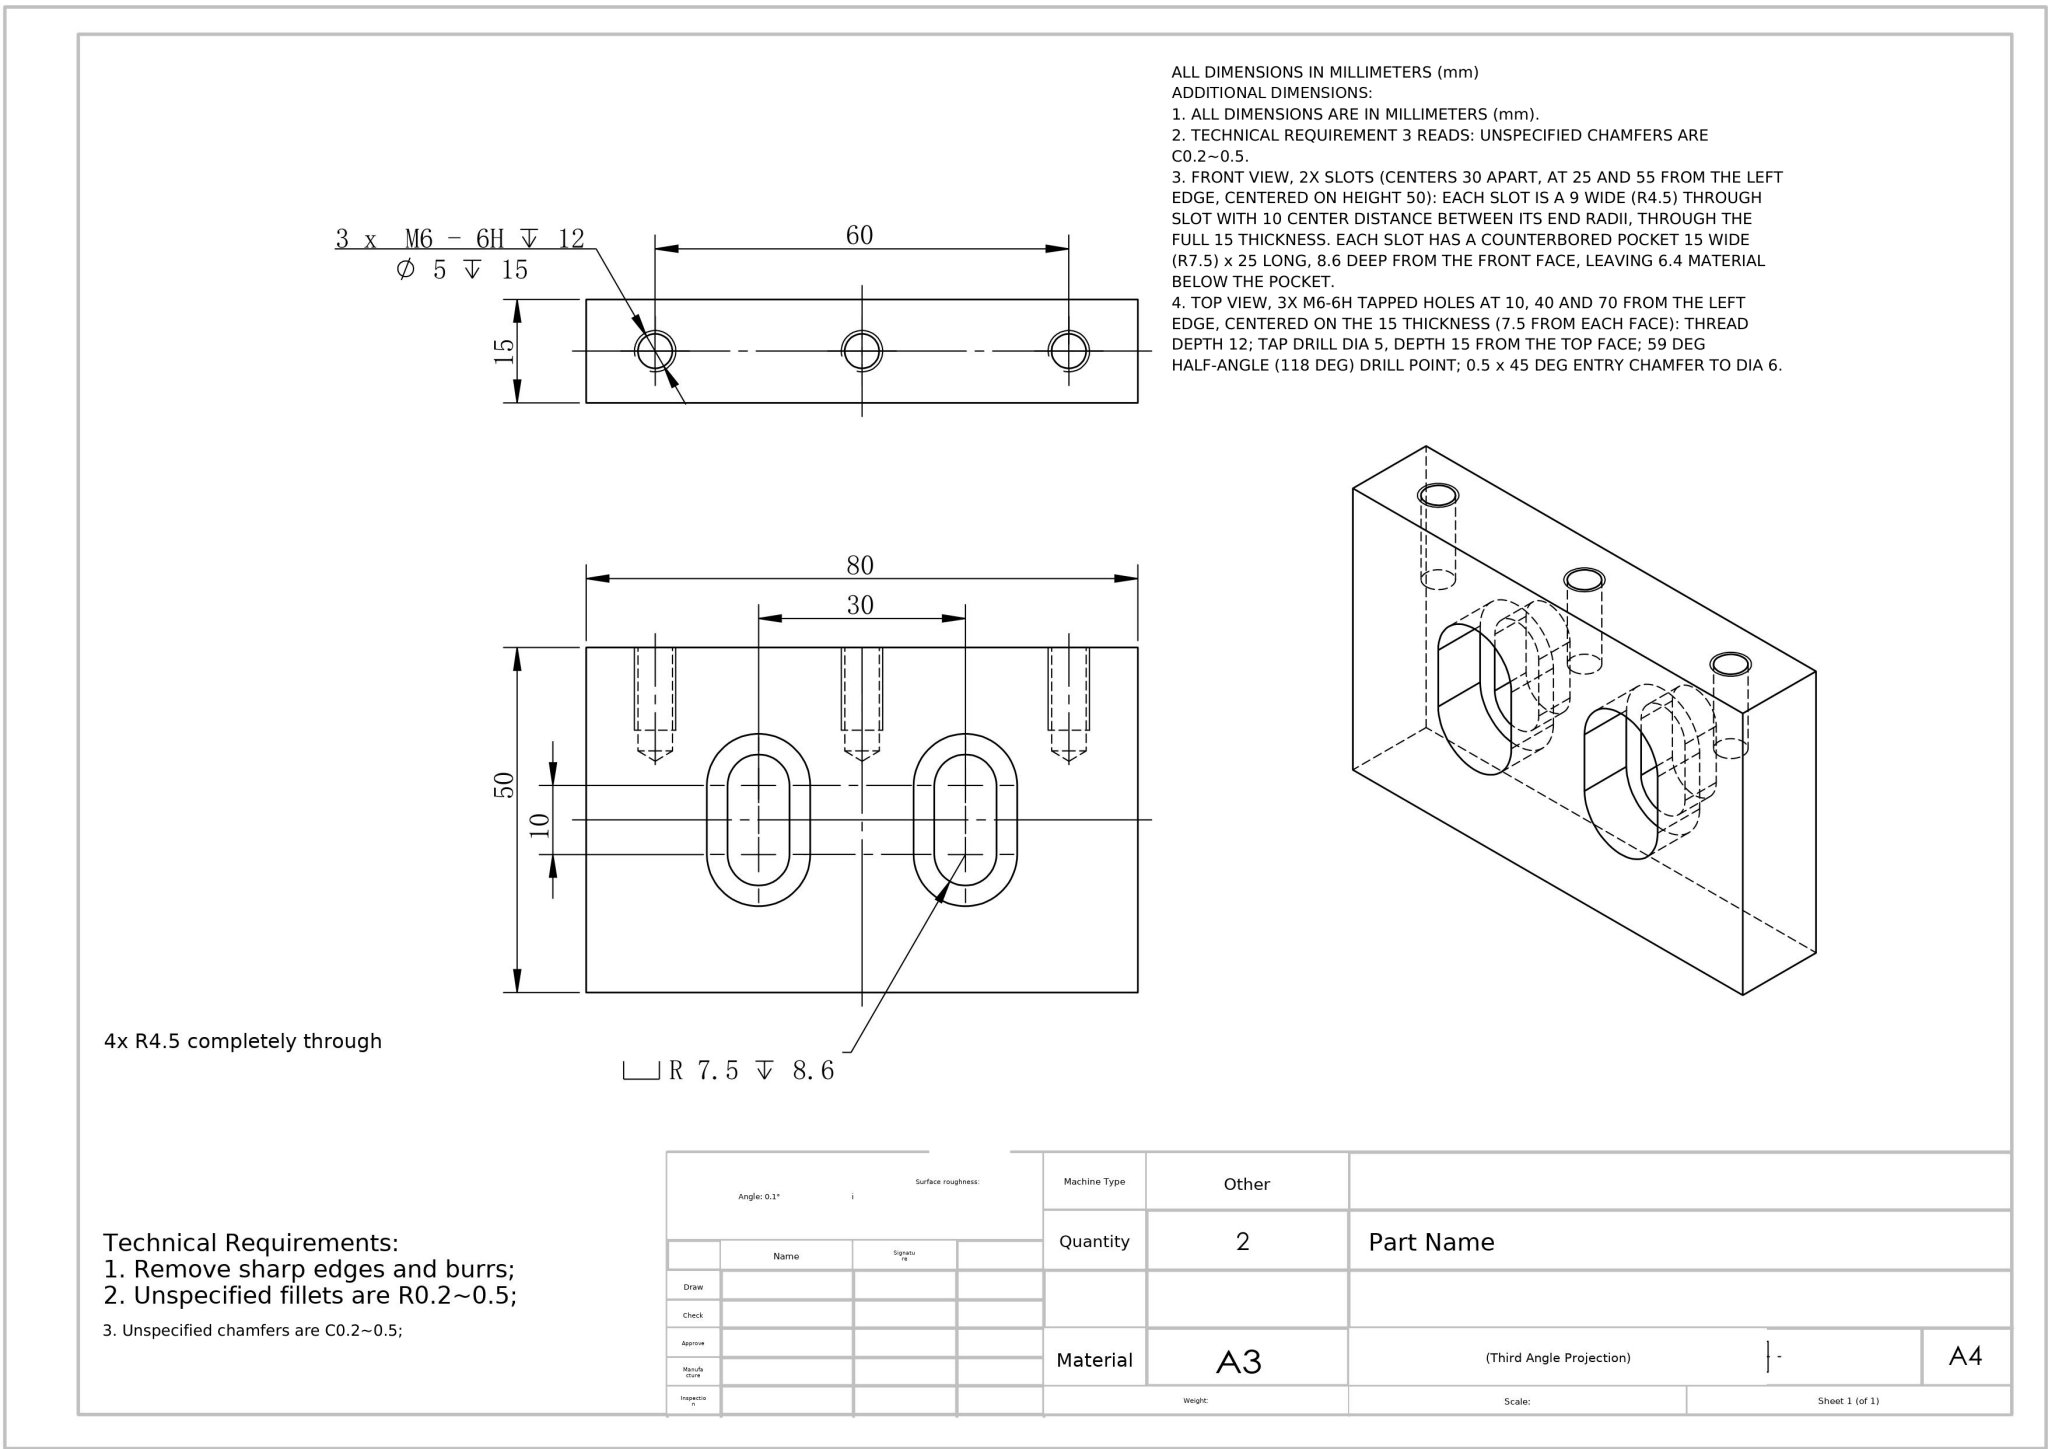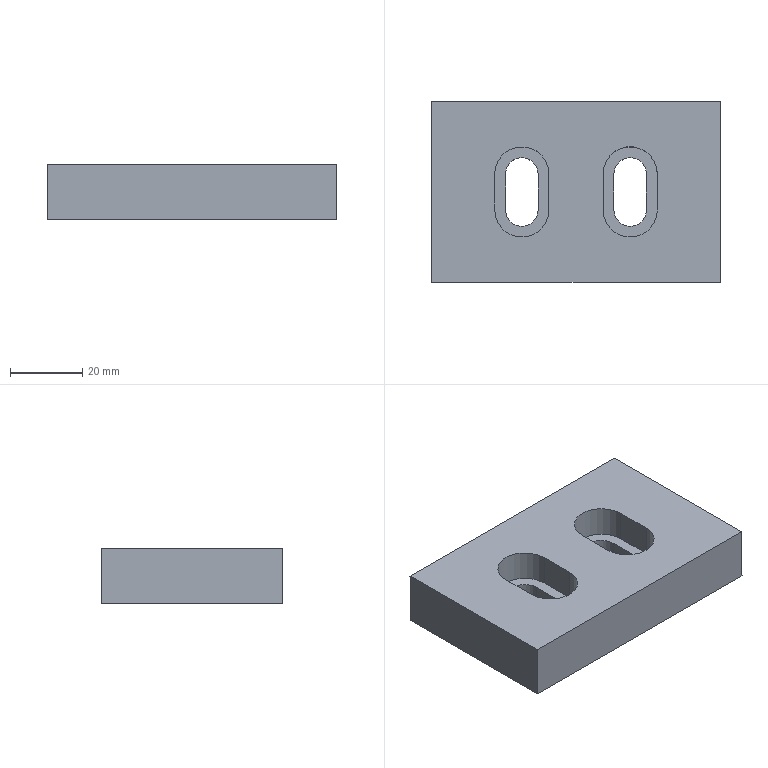Part | NX | mm | Dual Keyhole Mounting Plate | 1 solid | 33 faces | box 80.01 x 50.01 x 15 mm | volume 51495 mm3 | plane 16 | cylinder 11 | cone 6 | commonest cylinder face diameters 9 x4 15 x4 5 x3